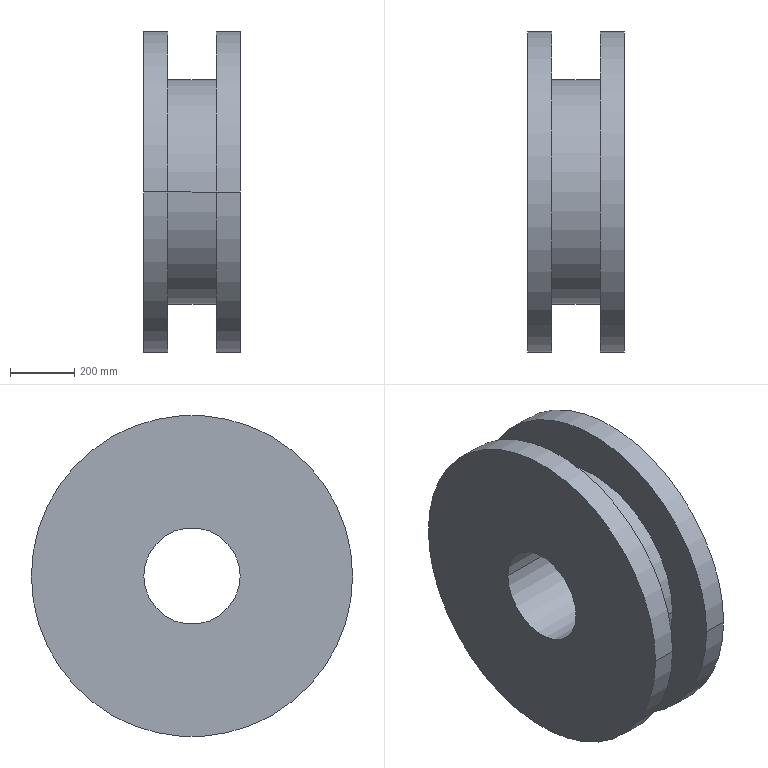Component | SolidWorks | LiftingAndOperatingMechanism-1_Part15-1 | 1 solid | 12 faces | box 300 x 1000 x 1000 mm | volume 154330739 mm3 | cylinder 8 | plane 4 | commonest cylinder face diameters 1000 x4 300 x2 700 x2
build123d program:
from build123d import *

# Parameters (mm, degrees)
SKETCH2_R          = 150
CUT_EXTRUDE1_DEPTH = 500


with BuildPart() as part:
    # Sketch1 → Revolve1 (revolve)
    with BuildSketch(Plane(origin=(0, 0, 0), x_dir=(0, 0, -1), z_dir=(1, 0, 0)), mode=Mode.PRIVATE) as revolve1_sk:
        Polygon((0, 0), (500, 0), (500, 75), (350, 75), (350, 225), (500, 225), (500, 300), (0, 300), align=None)
    revolve(revolve1_sk.sketch.rotate(Axis((0, 300, 0), (0, -1, 0)), 180), axis=Axis((0, 300, 0), (0, -1, 0)))

    # Sketch2 → Cut-Extrude1 (cut)
    with BuildSketch(Plane.XZ):
        with Locations(Location((0, 0, 0), (0, 0, 270))):
            Circle(SKETCH2_R)
    extrude(amount=-CUT_EXTRUDE1_DEPTH, mode=Mode.SUBTRACT)


solid = part.part

# Placed as in the assembly
solid = solid.moved(Location((3026.037, 13568.918, 4082.152), (0, 0, 90)))
STEP:
#1=COLOUR_RGB('',0.7922,0.8196,0.9333);
#2=FILL_AREA_STYLE_COLOUR('',#1);
#3=FILL_AREA_STYLE('',(#2));
#4=SURFACE_STYLE_FILL_AREA(#3);
#5=SURFACE_SIDE_STYLE('',(#4));
#6=SURFACE_STYLE_USAGE(.BOTH.,#5);
#7=PRESENTATION_STYLE_ASSIGNMENT((#6));
#8=CARTESIAN_POINT('',(107.324,540.115,160.715));
#9=VERTEX_POINT('',#8);
#10=CARTESIAN_POINT('',(107.324,528.304,160.715));
#11=VERTEX_POINT('',#10);
#12=CARTESIAN_POINT('',(107.324,534.209,160.715));
#13=DIRECTION('',(1.,0.,-0.0000002));
#14=DIRECTION('',(0.,-1.,0.));
#15=AXIS2_PLACEMENT_3D('',#12,#13,#14);
#16=CIRCLE('',#15,5.906);
#17=EDGE_CURVE('',#9,#11,#16,.T.);
#18=ORIENTED_EDGE('',*,*,#17,.F.);
#19=CARTESIAN_POINT('',(119.135,540.115,160.715));
#20=VERTEX_POINT('',#19);
#21=CARTESIAN_POINT('',(99.45,540.115,160.715));
#22=DIRECTION('',(1.,0.,-0.0000002));
#23=VECTOR('',#22,39.37);
#24=LINE('',#21,#23);
#25=EDGE_CURVE('',#9,#20,#24,.T.);
#26=ORIENTED_EDGE('',*,*,#25,.T.);
#27=CARTESIAN_POINT('',(119.135,528.304,160.715));
#28=VERTEX_POINT('',#27);
#29=CARTESIAN_POINT('',(119.135,534.209,160.715));
#30=DIRECTION('',(1.,0.,-0.0000002));
#31=DIRECTION('',(0.,-1.,0.));
#32=AXIS2_PLACEMENT_3D('',#29,#30,#31);
#33=CIRCLE('',#32,5.906);
#34=EDGE_CURVE('',#20,#28,#33,.T.);
#35=ORIENTED_EDGE('',*,*,#34,.T.);
#36=CARTESIAN_POINT('',(99.45,528.304,160.715));
#37=DIRECTION('',(1.,0.,-0.0000002));
#38=VECTOR('',#37,39.37);
#39=LINE('',#36,#38);
#40=EDGE_CURVE('',#11,#28,#39,.T.);
#41=ORIENTED_EDGE('',*,*,#40,.F.);
#42=EDGE_LOOP('',(#18,#26,#35,#41));
#43=FACE_OUTER_BOUND('',#42,.T.);
#44=CARTESIAN_POINT('',(99.45,534.209,160.715));
#45=DIRECTION('',(1.,0.,-0.0000002));
#46=DIRECTION('',(0.,-1.,0.));
#47=AXIS2_PLACEMENT_3D('',#44,#45,#46);
#48=CYLINDRICAL_SURFACE('',#47,5.906);
#49=ADVANCED_FACE('',(#43),#48,.F.);
#50=CARTESIAN_POINT('',(110.277,553.894,160.715));
#51=VERTEX_POINT('',#50);
#52=CARTESIAN_POINT('',(110.277,514.524,160.715));
#53=VERTEX_POINT('',#52);
#54=CARTESIAN_POINT('',(110.277,534.209,160.715));
#55=DIRECTION('',(-1.,-0.,0.0000002));
#56=DIRECTION('',(0.,1.,0.));
#57=AXIS2_PLACEMENT_3D('',#54,#55,#56);
#58=CIRCLE('',#57,19.685);
#59=EDGE_CURVE('',#51,#53,#58,.T.);
#60=ORIENTED_EDGE('',*,*,#59,.T.);
#61=CARTESIAN_POINT('',(107.324,514.524,160.715));
#62=VERTEX_POINT('',#61);
#63=CARTESIAN_POINT('',(107.324,514.524,160.715));
#64=DIRECTION('',(-1.,-0.,0.0000002));
#65=VECTOR('',#64,39.37);
#66=LINE('',#63,#65);
#67=EDGE_CURVE('',#53,#62,#66,.T.);
#68=ORIENTED_EDGE('',*,*,#67,.T.);
#69=CARTESIAN_POINT('',(107.324,553.894,160.715));
#70=VERTEX_POINT('',#69);
#71=CARTESIAN_POINT('',(107.324,534.209,160.715));
#72=DIRECTION('',(-1.,-0.,0.0000002));
#73=DIRECTION('',(0.,1.,0.));
#74=AXIS2_PLACEMENT_3D('',#71,#72,#73);
#75=CIRCLE('',#74,19.685);
#76=EDGE_CURVE('',#70,#62,#75,.T.);
#77=ORIENTED_EDGE('',*,*,#76,.F.);
#78=CARTESIAN_POINT('',(107.324,553.894,160.715));
#79=DIRECTION('',(-1.,-0.,0.0000002));
#80=VECTOR('',#79,39.37);
#81=LINE('',#78,#80);
#82=EDGE_CURVE('',#51,#70,#81,.T.);
#83=ORIENTED_EDGE('',*,*,#82,.F.);
#84=EDGE_LOOP('',(#60,#68,#77,#83));
#85=FACE_OUTER_BOUND('',#84,.T.);
#86=CARTESIAN_POINT('',(107.324,534.209,160.715));
#87=DIRECTION('',(-1.,-0.,0.0000002));
#88=DIRECTION('',(0.,1.,0.));
#89=AXIS2_PLACEMENT_3D('',#86,#87,#88);
#90=CYLINDRICAL_SURFACE('',#89,19.685);
#91=ADVANCED_FACE('',(#85),#90,.T.);
#92=CARTESIAN_POINT('',(116.183,547.989,160.715));
#93=VERTEX_POINT('',#92);
#94=CARTESIAN_POINT('',(116.183,520.43,160.715));
#95=VERTEX_POINT('',#94);
#96=CARTESIAN_POINT('',(116.183,534.209,160.715));
#97=DIRECTION('',(-1.,-0.,0.0000002));
#98=DIRECTION('',(0.,1.,0.));
#99=AXIS2_PLACEMENT_3D('',#96,#97,#98);
#100=CIRCLE('',#99,13.78);
#101=EDGE_CURVE('',#93,#95,#100,.T.);
#102=ORIENTED_EDGE('',*,*,#101,.T.);
#103=CARTESIAN_POINT('',(110.277,520.43,160.715));
#104=VERTEX_POINT('',#103);
#105=CARTESIAN_POINT('',(107.324,520.43,160.715));
#106=DIRECTION('',(-1.,-0.,0.0000002));
#107=VECTOR('',#106,39.37);
#108=LINE('',#105,#107);
#109=EDGE_CURVE('',#95,#104,#108,.T.);
#110=ORIENTED_EDGE('',*,*,#109,.T.);
#111=CARTESIAN_POINT('',(110.277,547.989,160.715));
#112=VERTEX_POINT('',#111);
#113=CARTESIAN_POINT('',(110.277,534.209,160.715));
#114=DIRECTION('',(-1.,-0.,0.0000002));
#115=DIRECTION('',(0.,1.,0.));
#116=AXIS2_PLACEMENT_3D('',#113,#114,#115);
#117=CIRCLE('',#116,13.78);
#118=EDGE_CURVE('',#112,#104,#117,.T.);
#119=ORIENTED_EDGE('',*,*,#118,.F.);
#120=CARTESIAN_POINT('',(107.324,547.989,160.715));
#121=DIRECTION('',(-1.,-0.,0.0000002));
#122=VECTOR('',#121,39.37);
#123=LINE('',#120,#122);
#124=EDGE_CURVE('',#93,#112,#123,.T.);
#125=ORIENTED_EDGE('',*,*,#124,.F.);
#126=EDGE_LOOP('',(#102,#110,#119,#125));
#127=FACE_OUTER_BOUND('',#126,.T.);
#128=CARTESIAN_POINT('',(107.324,534.209,160.715));
#129=DIRECTION('',(-1.,-0.,0.0000002));
#130=DIRECTION('',(0.,1.,0.));
#131=AXIS2_PLACEMENT_3D('',#128,#129,#130);
#132=CYLINDRICAL_SURFACE('',#131,13.78);
#133=ADVANCED_FACE('',(#127),#132,.T.);
#134=CARTESIAN_POINT('',(119.135,553.894,160.715));
#135=VERTEX_POINT('',#134);
#136=CARTESIAN_POINT('',(119.135,514.524,160.715));
#137=VERTEX_POINT('',#136);
#138=CARTESIAN_POINT('',(119.135,534.209,160.715));
#139=DIRECTION('',(-1.,-0.,0.0000002));
#140=DIRECTION('',(0.,1.,0.));
#141=AXIS2_PLACEMENT_3D('',#138,#139,#140);
#142=CIRCLE('',#141,19.685);
#143=EDGE_CURVE('',#135,#137,#142,.T.);
#144=ORIENTED_EDGE('',*,*,#143,.T.);
#145=CARTESIAN_POINT('',(116.183,514.524,160.715));
#146=VERTEX_POINT('',#145);
#147=CARTESIAN_POINT('',(107.324,514.524,160.715));
#148=DIRECTION('',(-1.,-0.,0.0000002));
#149=VECTOR('',#148,39.37);
#150=LINE('',#147,#149);
#151=EDGE_CURVE('',#137,#146,#150,.T.);
#152=ORIENTED_EDGE('',*,*,#151,.T.);
#153=CARTESIAN_POINT('',(116.183,553.894,160.715));
#154=VERTEX_POINT('',#153);
#155=CARTESIAN_POINT('',(116.183,534.209,160.715));
#156=DIRECTION('',(-1.,-0.,0.0000002));
#157=DIRECTION('',(0.,1.,0.));
#158=AXIS2_PLACEMENT_3D('',#155,#156,#157);
#159=CIRCLE('',#158,19.685);
#160=EDGE_CURVE('',#154,#146,#159,.T.);
#161=ORIENTED_EDGE('',*,*,#160,.F.);
#162=CARTESIAN_POINT('',(107.324,553.894,160.715));
#163=DIRECTION('',(-1.,-0.,0.0000002));
#164=VECTOR('',#163,39.37);
#165=LINE('',#162,#164);
#166=EDGE_CURVE('',#135,#154,#165,.T.);
#167=ORIENTED_EDGE('',*,*,#166,.F.);
#168=EDGE_LOOP('',(#144,#152,#161,#167));
#169=FACE_OUTER_BOUND('',#168,.T.);
#170=CARTESIAN_POINT('',(107.324,534.209,160.715));
#171=DIRECTION('',(-1.,-0.,0.0000002));
#172=DIRECTION('',(0.,1.,0.));
#173=AXIS2_PLACEMENT_3D('',#170,#171,#172);
#174=CYLINDRICAL_SURFACE('',#173,19.685);
#175=ADVANCED_FACE('',(#169),#174,.T.);
#176=CARTESIAN_POINT('',(119.135,534.209,160.715));
#177=DIRECTION('',(1.,0.,-0.0000002));
#178=DIRECTION('',(0.,-1.,0.));
#179=AXIS2_PLACEMENT_3D('',#176,#177,#178);
#180=CIRCLE('',#179,5.906);
#181=EDGE_CURVE('',#28,#20,#180,.T.);
#182=ORIENTED_EDGE('',*,*,#181,.F.);
#183=ORIENTED_EDGE('',*,*,#34,.F.);
#184=EDGE_LOOP('',(#182,#183));
#185=FACE_BOUND('',#184,.T.);
#186=ORIENTED_EDGE('',*,*,#143,.F.);
#187=CARTESIAN_POINT('',(119.135,534.209,160.715));
#188=DIRECTION('',(-1.,-0.,0.0000002));
#189=DIRECTION('',(0.,1.,0.));
#190=AXIS2_PLACEMENT_3D('',#187,#188,#189);
#191=CIRCLE('',#190,19.685);
#192=EDGE_CURVE('',#137,#135,#191,.T.);
#193=ORIENTED_EDGE('',*,*,#192,.F.);
#194=EDGE_LOOP('',(#186,#193));
#195=FACE_OUTER_BOUND('',#194,.T.);
#196=CARTESIAN_POINT('',(119.135,534.209,160.715));
#197=DIRECTION('',(-1.,-0.,0.0000002));
#198=DIRECTION('',(-0.,1.,0.));
#199=AXIS2_PLACEMENT_3D('',#196,#197,#198);
#200=PLANE('',#199);
#201=ADVANCED_FACE('',(#185,#195),#200,.F.);
#202=ORIENTED_EDGE('',*,*,#151,.F.);
#203=ORIENTED_EDGE('',*,*,#192,.T.);
#204=ORIENTED_EDGE('',*,*,#166,.T.);
#205=CARTESIAN_POINT('',(116.183,534.209,160.715));
#206=DIRECTION('',(-1.,-0.,0.0000002));
#207=DIRECTION('',(0.,1.,0.));
#208=AXIS2_PLACEMENT_3D('',#205,#206,#207);
#209=CIRCLE('',#208,19.685);
#210=EDGE_CURVE('',#146,#154,#209,.T.);
#211=ORIENTED_EDGE('',*,*,#210,.F.);
#212=EDGE_LOOP('',(#202,#203,#204,#211));
#213=FACE_OUTER_BOUND('',#212,.T.);
#214=CARTESIAN_POINT('',(107.324,534.209,160.715));
#215=DIRECTION('',(-1.,-0.,0.0000002));
#216=DIRECTION('',(0.,1.,0.));
#217=AXIS2_PLACEMENT_3D('',#214,#215,#216);
#218=CYLINDRICAL_SURFACE('',#217,19.685);
#219=ADVANCED_FACE('',(#213),#218,.T.);
#220=ORIENTED_EDGE('',*,*,#101,.F.);
#221=CARTESIAN_POINT('',(116.183,534.209,160.715));
#222=DIRECTION('',(-1.,-0.,0.0000002));
#223=DIRECTION('',(0.,1.,0.));
#224=AXIS2_PLACEMENT_3D('',#221,#222,#223);
#225=CIRCLE('',#224,13.78);
#226=EDGE_CURVE('',#95,#93,#225,.T.);
#227=ORIENTED_EDGE('',*,*,#226,.F.);
#228=EDGE_LOOP('',(#220,#227));
#229=FACE_BOUND('',#228,.T.);
#230=ORIENTED_EDGE('',*,*,#160,.T.);
#231=ORIENTED_EDGE('',*,*,#210,.T.);
#232=EDGE_LOOP('',(#230,#231));
#233=FACE_OUTER_BOUND('',#232,.T.);
#234=CARTESIAN_POINT('',(116.183,514.524,160.715));
#235=DIRECTION('',(1.,0.,-0.0000002));
#236=DIRECTION('',(0.,-1.,-0.));
#237=AXIS2_PLACEMENT_3D('',#234,#235,#236);
#238=PLANE('',#237);
#239=ADVANCED_FACE('',(#229,#233),#238,.F.);
#240=ORIENTED_EDGE('',*,*,#109,.F.);
#241=ORIENTED_EDGE('',*,*,#226,.T.);
#242=ORIENTED_EDGE('',*,*,#124,.T.);
#243=CARTESIAN_POINT('',(110.277,534.209,160.715));
#244=DIRECTION('',(-1.,-0.,0.0000002));
#245=DIRECTION('',(0.,1.,0.));
#246=AXIS2_PLACEMENT_3D('',#243,#244,#245);
#247=CIRCLE('',#246,13.78);
#248=EDGE_CURVE('',#104,#112,#247,.T.);
#249=ORIENTED_EDGE('',*,*,#248,.F.);
#250=EDGE_LOOP('',(#240,#241,#242,#249));
#251=FACE_OUTER_BOUND('',#250,.T.);
#252=CARTESIAN_POINT('',(107.324,534.209,160.715));
#253=DIRECTION('',(-1.,-0.,0.0000002));
#254=DIRECTION('',(0.,1.,0.));
#255=AXIS2_PLACEMENT_3D('',#252,#253,#254);
#256=CYLINDRICAL_SURFACE('',#255,13.78);
#257=ADVANCED_FACE('',(#251),#256,.T.);
#258=ORIENTED_EDGE('',*,*,#59,.F.);
#259=CARTESIAN_POINT('',(110.277,534.209,160.715));
#260=DIRECTION('',(-1.,-0.,0.0000002));
#261=DIRECTION('',(0.,1.,0.));
#262=AXIS2_PLACEMENT_3D('',#259,#260,#261);
#263=CIRCLE('',#262,19.685);
#264=EDGE_CURVE('',#53,#51,#263,.T.);
#265=ORIENTED_EDGE('',*,*,#264,.F.);
#266=EDGE_LOOP('',(#258,#265));
#267=FACE_OUTER_BOUND('',#266,.T.);
#268=ORIENTED_EDGE('',*,*,#118,.T.);
#269=ORIENTED_EDGE('',*,*,#248,.T.);
#270=EDGE_LOOP('',(#268,#269));
#271=FACE_BOUND('',#270,.T.);
#272=CARTESIAN_POINT('',(110.277,520.43,160.715));
#273=DIRECTION('',(-1.,-0.,0.0000002));
#274=DIRECTION('',(-0.,1.,0.));
#275=AXIS2_PLACEMENT_3D('',#272,#273,#274);
#276=PLANE('',#275);
#277=ADVANCED_FACE('',(#267,#271),#276,.F.);
#278=ORIENTED_EDGE('',*,*,#67,.F.);
#279=ORIENTED_EDGE('',*,*,#264,.T.);
#280=ORIENTED_EDGE('',*,*,#82,.T.);
#281=CARTESIAN_POINT('',(107.324,534.209,160.715));
#282=DIRECTION('',(-1.,-0.,0.0000002));
#283=DIRECTION('',(0.,1.,0.));
#284=AXIS2_PLACEMENT_3D('',#281,#282,#283);
#285=CIRCLE('',#284,19.685);
#286=EDGE_CURVE('',#62,#70,#285,.T.);
#287=ORIENTED_EDGE('',*,*,#286,.F.);
#288=EDGE_LOOP('',(#278,#279,#280,#287));
#289=FACE_OUTER_BOUND('',#288,.T.);
#290=CARTESIAN_POINT('',(107.324,534.209,160.715));
#291=DIRECTION('',(-1.,-0.,0.0000002));
#292=DIRECTION('',(0.,1.,0.));
#293=AXIS2_PLACEMENT_3D('',#290,#291,#292);
#294=CYLINDRICAL_SURFACE('',#293,19.685);
#295=ADVANCED_FACE('',(#289),#294,.T.);
#296=CARTESIAN_POINT('',(107.324,534.209,160.715));
#297=DIRECTION('',(1.,0.,-0.0000002));
#298=DIRECTION('',(0.,-1.,0.));
#299=AXIS2_PLACEMENT_3D('',#296,#297,#298);
#300=CIRCLE('',#299,5.906);
#301=EDGE_CURVE('',#11,#9,#300,.T.);
#302=ORIENTED_EDGE('',*,*,#301,.T.);
#303=ORIENTED_EDGE('',*,*,#17,.T.);
#304=EDGE_LOOP('',(#302,#303));
#305=FACE_BOUND('',#304,.T.);
#306=ORIENTED_EDGE('',*,*,#76,.T.);
#307=ORIENTED_EDGE('',*,*,#286,.T.);
#308=EDGE_LOOP('',(#306,#307));
#309=FACE_OUTER_BOUND('',#308,.T.);
#310=CARTESIAN_POINT('',(107.324,514.524,160.715));
#311=DIRECTION('',(1.,0.,-0.0000002));
#312=DIRECTION('',(0.,-1.,-0.));
#313=AXIS2_PLACEMENT_3D('',#310,#311,#312);
#314=PLANE('',#313);
#315=ADVANCED_FACE('',(#305,#309),#314,.F.);
#316=ORIENTED_EDGE('',*,*,#25,.F.);
#317=ORIENTED_EDGE('',*,*,#301,.F.);
#318=ORIENTED_EDGE('',*,*,#40,.T.);
#319=ORIENTED_EDGE('',*,*,#181,.T.);
#320=EDGE_LOOP('',(#316,#317,#318,#319));
#321=FACE_OUTER_BOUND('',#320,.T.);
#322=CARTESIAN_POINT('',(99.45,534.209,160.715));
#323=DIRECTION('',(1.,0.,-0.0000002));
#324=DIRECTION('',(0.,-1.,0.));
#325=AXIS2_PLACEMENT_3D('',#322,#323,#324);
#326=CYLINDRICAL_SURFACE('',#325,5.906);
#327=ADVANCED_FACE('',(#321),#326,.F.);
#328=CLOSED_SHELL('',(#49,#91,#133,#175,#201,#219,#239,#257,#277,#295,#315,#327));
#329=MANIFOLD_SOLID_BREP('',#328);
#330=STYLED_ITEM('',(#7),#329);
#331=PRESENTATION_LAYER_ASSIGNMENT('','',(#330));
#332=CARTESIAN_POINT('',(0.,0.,0.));
#333=DIRECTION('',(0.,0.,1.));
#334=DIRECTION('',(1.,0.,0.));
#335=AXIS2_PLACEMENT_3D('',#332,#333,#334);
#336=(LENGTH_UNIT()NAMED_UNIT(*)SI_UNIT($,.METRE.));
#337=LENGTH_MEASURE_WITH_UNIT(LENGTH_MEASURE(0.0254),#336);
#338=DIMENSIONAL_EXPONENTS(1.,0.,0.,0.,0.,0.,0.);
#339=(CONVERSION_BASED_UNIT('',#337)LENGTH_UNIT()NAMED_UNIT(#338));
#340=UNCERTAINTY_MEASURE_WITH_UNIT(LENGTH_MEASURE(0.00001),#339,'','');
#341=(NAMED_UNIT(*)PLANE_ANGLE_UNIT()SI_UNIT($,.RADIAN.));
#342=(NAMED_UNIT(*)SI_UNIT($,.STERADIAN.)SOLID_ANGLE_UNIT());
#343=(GEOMETRIC_REPRESENTATION_CONTEXT(3)GLOBAL_UNCERTAINTY_ASSIGNED_CONTEXT((#340))GLOBAL_UNIT_ASSIGNED_CONTEXT((#339,#341,#342))REPRESENTATION_CONTEXT('',''));
#344=ADVANCED_BREP_SHAPE_REPRESENTATION('',(#329,#335),#343);
#345=(LENGTH_UNIT()NAMED_UNIT(*)SI_UNIT($,.METRE.));
#346=LENGTH_MEASURE_WITH_UNIT(LENGTH_MEASURE(0.0254),#345);
#347=DIMENSIONAL_EXPONENTS(1.,0.,0.,0.,0.,0.,0.);
#348=(CONVERSION_BASED_UNIT('',#346)LENGTH_UNIT()NAMED_UNIT(#347));
#349=UNCERTAINTY_MEASURE_WITH_UNIT(LENGTH_MEASURE(0.00001),#348,'','');
#350=(NAMED_UNIT(*)PLANE_ANGLE_UNIT()SI_UNIT($,.RADIAN.));
#351=(NAMED_UNIT(*)SI_UNIT($,.STERADIAN.)SOLID_ANGLE_UNIT());
#352=(GEOMETRIC_REPRESENTATION_CONTEXT(3)GLOBAL_UNCERTAINTY_ASSIGNED_CONTEXT((#349))GLOBAL_UNIT_ASSIGNED_CONTEXT((#348,#350,#351))REPRESENTATION_CONTEXT('',''));
#353=MECHANICAL_DESIGN_GEOMETRIC_PRESENTATION_REPRESENTATION('',(#330),#352);